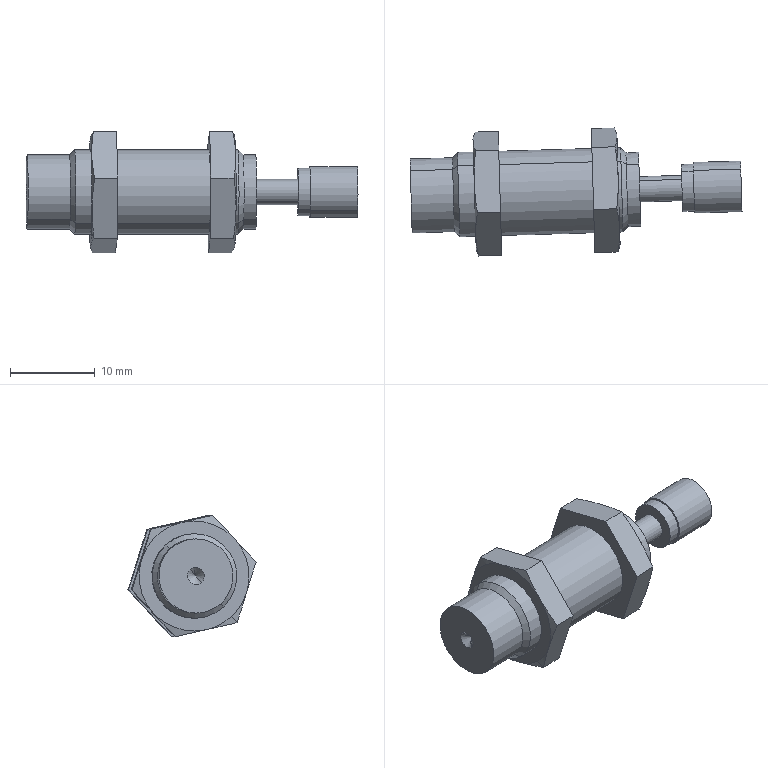Component | SolidWorks | BufferMAKC1005A-1 | 4 solids | 61 faces | volume 2545 mm3 | plane 23 | cone 20 | cylinder 18 | commonest cylinder face diameters 10.002 x4 3 x4 8.773 x4 5.6 x2 6 x2 10 x2 | material Standard Parts